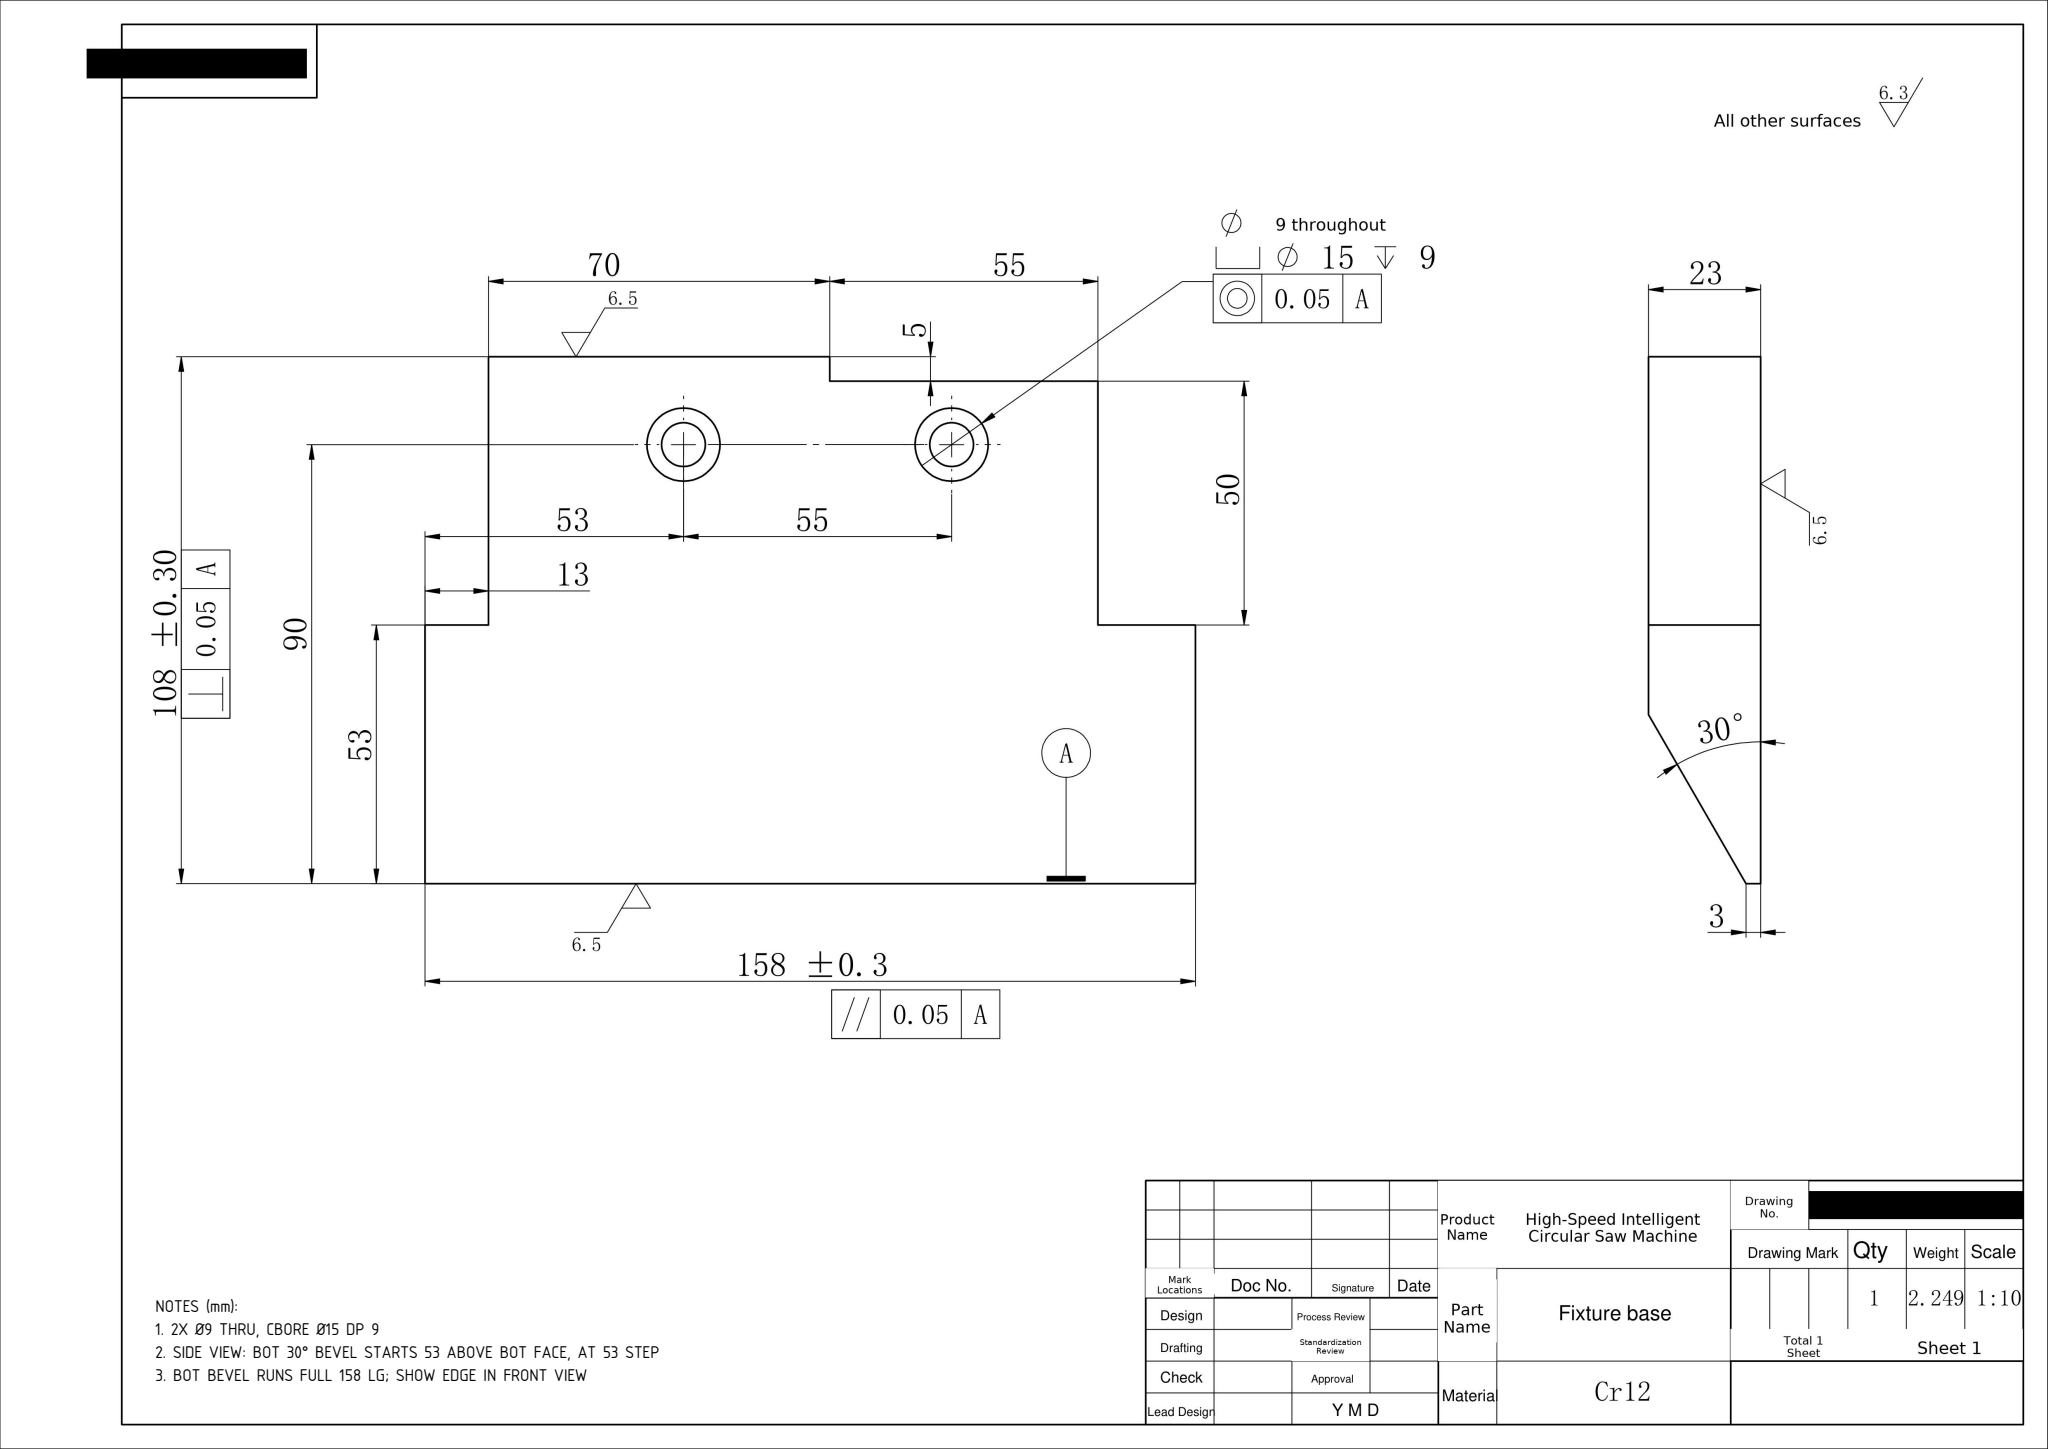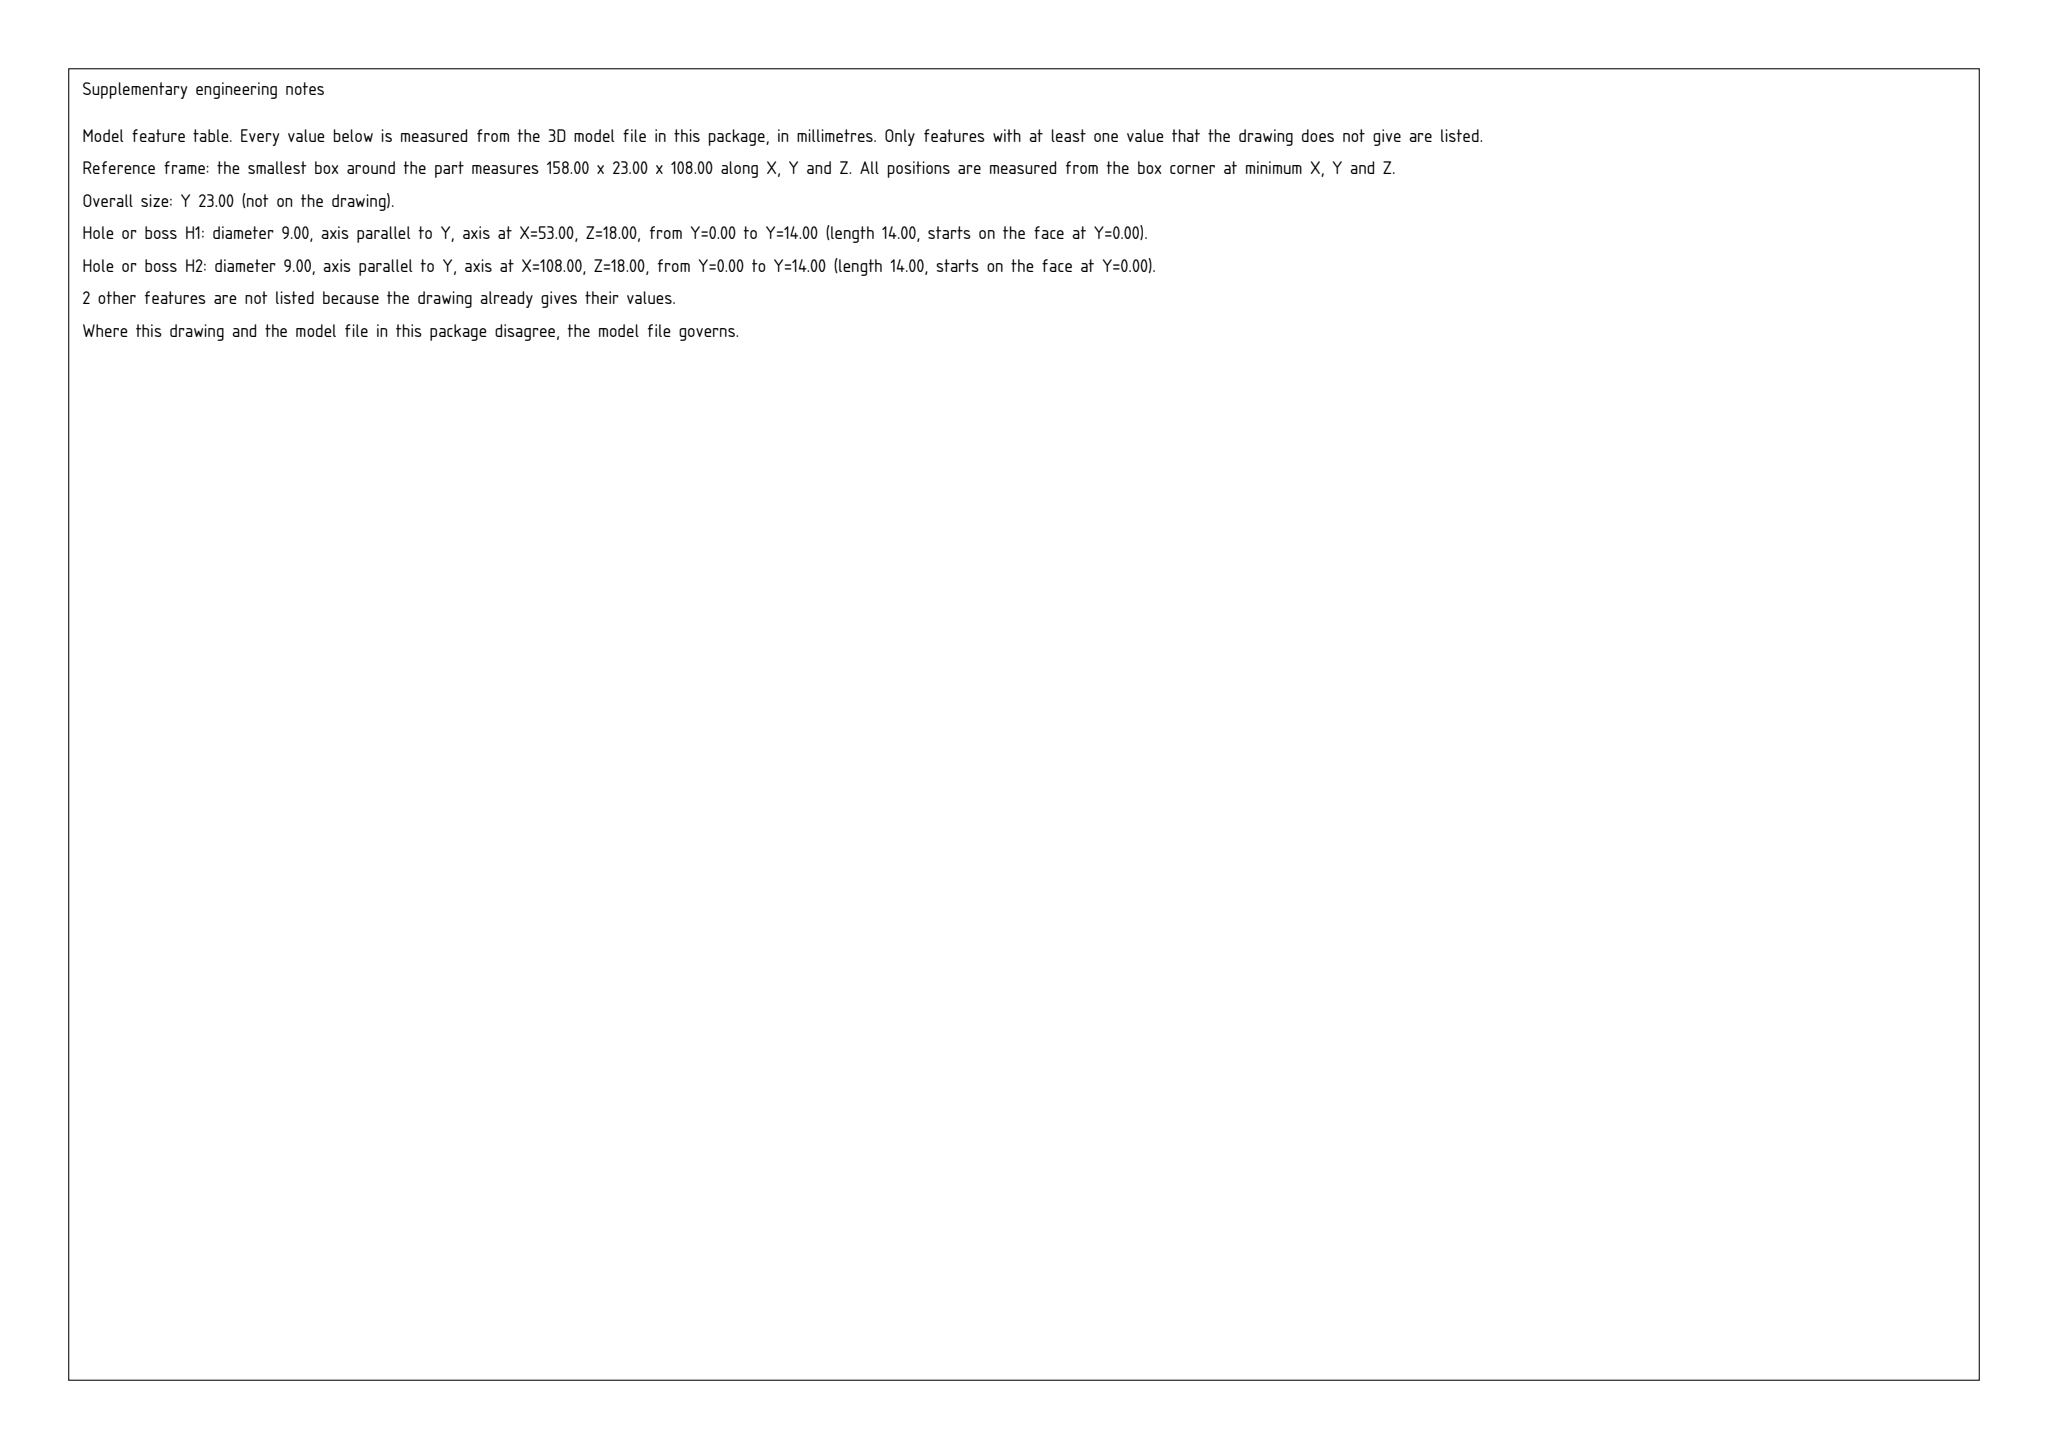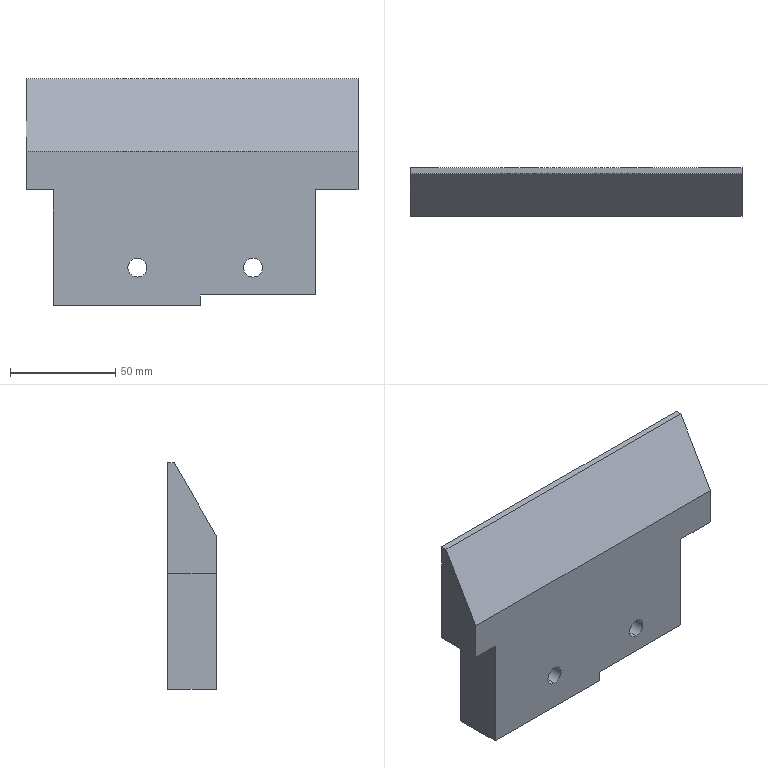Part | SolidWorks | mm | 1 solid | 23 faces | box 158 x 23 x 108 mm | volume 284707 mm3 | plane 15 | cylinder 8 | commonest cylinder face diameters 15 x4 9 x4
Drawing notes:
2X Ø9 THRU, CBORE Ø15 DP 9 | from the solid: Ø9 y-axis holes at x=53 & x=108 (55 apart), z=18; Ø15 c'bores 9 deep at same axes
SIDE VIEW: BOT 30° BEVEL STARTS 53 ABOVE BOT FACE, AT 53 STEP | from the solid: z-planes at 0,5,55,108; bevel start edge at z=55 (2 faces) = 108-55 = 53 from bottom face (z=108); matches front-view 53 step
BOT BEVEL RUNS FULL 158 LG; SHOW EDGE IN FRONT VIEW | from the solid: x-planes only at 0,13,83,138,158; no intermediate x boundary limits bevel, so it spans full 158 bbox length
build123d program:
from build123d import *

# Parameters (mm, degrees)
SKETCH2_W                                          = 125
SKETCH2_H                                          = 23
BOSS_EXTRUDE1_DEPTH                                = 210
SKETCH4_W                                          = 127
SKETCH4_H                                          = 23
CUT_EXTRUDE2_DEPTH                                 = 7
CUT_EXTRUDE3_DEPTH                                 = 234.728
SKETCH12_W                                         = 68
SKETCH12_H                                         = 28
CUT_EXTRUDE4_DEPTH                                 = 2
HOLE_SIZE_ACCORDING_TO_THE_TYPE_OF_HEX_D           = 9
HOLE_SIZE_ACCORDING_TO_THE_TYPE_OF_HEX_CBORE_D     = 15
HOLE_SIZE_ACCORDING_TO_THE_TYPE_OF_HEX_CBORE_DEPTH = 9
CUT_EXTRUDE5_DEPTH                                 = 86


with BuildPart() as part:
    # Sketch2 → Boss-Extrude1 (new body)
    with BuildSketch(Plane(origin=(0, 0, 0), x_dir=(0, 0, -1), z_dir=(1, 0, 0))):
        with Locations((37.5, 11.5)):
            Rectangle(SKETCH2_W, SKETCH2_H)
    extrude(amount=-BOSS_EXTRUDE1_DEPTH)

    # Sketch4 → Cut-Extrude2 (cut)
    with BuildSketch(Plane(origin=(0, 0, -100), x_dir=(-1, 0, 0), z_dir=(0, 0, -1))):
        with Locations((63.5, 11.5)):
            Rectangle(SKETCH4_W, SKETCH4_H)
    extrude(amount=-CUT_EXTRUDE2_DEPTH, mode=Mode.SUBTRACT)

    # Sketch9 → Cut-Extrude3 (cut, through all)
    with BuildSketch(Plane(origin=(0, 0, 0), x_dir=(0, 0, -1), z_dir=(1, 0, 0))):
        Polygon((-25, 23), (-25, 0), (24.641, 0), (-10, 20), (-10, 23), align=None)
    extrude(amount=-CUT_EXTRUDE3_DEPTH, mode=Mode.SUBTRACT)

    # Sketch12 → Cut-Extrude4 (cut)
    with BuildSketch(Plane(origin=(0, 0, -100), x_dir=(-1, 0, 0), z_dir=(0, 0, -1))):
        with Locations((161, 14)):
            Rectangle(SKETCH12_W, SKETCH12_H)
    extrude(amount=-CUT_EXTRUDE4_DEPTH, mode=Mode.SUBTRACT)

    # Hole Size _according to_ the type of Hex (through all)
    with Locations(Plane(origin=(0, 23, 0), x_dir=(1, 0, 0), z_dir=(0, 1, 0))):
        with Locations((-157, 80), (-102, 80)):
            CounterBoreHole(HOLE_SIZE_ACCORDING_TO_THE_TYPE_OF_HEX_D / 2, HOLE_SIZE_ACCORDING_TO_THE_TYPE_OF_HEX_CBORE_D / 2, HOLE_SIZE_ACCORDING_TO_THE_TYPE_OF_HEX_CBORE_DEPTH)

    # Sketch16 → Cut-Extrude5 (cut)
    with BuildSketch(Plane(origin=(0, 23, 0), x_dir=(1, 0, 0), z_dir=(0, 1, 0))):
        Polygon((-197, 98), (-197, 43), (-210, 43), (-210, 100), (-195, 100), (-195, 98), align=None)
        Polygon((-52, 43), (-52, -25), (0, -25), (0, 43), (26.134, 43), (26.134, 98), (-72, 98), (-72, 43), align=None)
    extrude(amount=-CUT_EXTRUDE5_DEPTH, mode=Mode.SUBTRACT)


solid = part.part
STEP:
#1=CARTESIAN_POINT('',(-157.,14.,-87.5));
#2=VERTEX_POINT('',#1);
#3=CARTESIAN_POINT('',(-157.,14.,-72.5));
#4=VERTEX_POINT('',#3);
#5=CARTESIAN_POINT('',(-157.,14.,-80.));
#6=DIRECTION('',(0.,1.,0.));
#7=DIRECTION('',(0.,-0.,1.));
#8=AXIS2_PLACEMENT_3D('',#5,#6,#7);
#9=CIRCLE('',#8,7.5);
#10=EDGE_CURVE('',#2,#4,#9,.T.);
#11=ORIENTED_EDGE('',*,*,#10,.F.);
#12=CARTESIAN_POINT('',(-157.,23.,-87.5));
#13=VERTEX_POINT('',#12);
#14=CARTESIAN_POINT('',(-157.,23.,-87.5));
#15=DIRECTION('',(0.,1.,0.));
#16=VECTOR('',#15,1000.);
#17=LINE('',#14,#16);
#18=EDGE_CURVE('',#2,#13,#17,.T.);
#19=ORIENTED_EDGE('',*,*,#18,.T.);
#20=CARTESIAN_POINT('',(-157.,23.,-72.5));
#21=VERTEX_POINT('',#20);
#22=CARTESIAN_POINT('',(-157.,23.,-80.));
#23=DIRECTION('',(0.,1.,0.));
#24=DIRECTION('',(0.,0.,1.));
#25=AXIS2_PLACEMENT_3D('',#22,#23,#24);
#26=CIRCLE('',#25,7.5);
#27=EDGE_CURVE('',#13,#21,#26,.T.);
#28=ORIENTED_EDGE('',*,*,#27,.T.);
#29=CARTESIAN_POINT('',(-157.,23.,-72.5));
#30=DIRECTION('',(0.,1.,0.));
#31=VECTOR('',#30,1000.);
#32=LINE('',#29,#31);
#33=EDGE_CURVE('',#4,#21,#32,.T.);
#34=ORIENTED_EDGE('',*,*,#33,.F.);
#35=EDGE_LOOP('',(#11,#19,#28,#34));
#36=FACE_OUTER_BOUND('',#35,.T.);
#37=CARTESIAN_POINT('',(-157.,23.,-80.));
#38=DIRECTION('',(0.,1.,0.));
#39=DIRECTION('',(0.,0.,1.));
#40=AXIS2_PLACEMENT_3D('',#37,#38,#39);
#41=CYLINDRICAL_SURFACE('',#40,7.5);
#42=ADVANCED_FACE('',(#36),#41,.F.);
#43=CARTESIAN_POINT('',(-157.,-0.,-84.5));
#44=VERTEX_POINT('',#43);
#45=CARTESIAN_POINT('',(-157.,-0.,-75.5));
#46=VERTEX_POINT('',#45);
#47=CARTESIAN_POINT('',(-157.,-0.,-80.));
#48=DIRECTION('',(0.,1.,0.));
#49=DIRECTION('',(0.,-0.,1.));
#50=AXIS2_PLACEMENT_3D('',#47,#48,#49);
#51=CIRCLE('',#50,4.5);
#52=EDGE_CURVE('',#44,#46,#51,.T.);
#53=ORIENTED_EDGE('',*,*,#52,.F.);
#54=CARTESIAN_POINT('',(-157.,14.,-84.5));
#55=VERTEX_POINT('',#54);
#56=CARTESIAN_POINT('',(-157.,23.,-84.5));
#57=DIRECTION('',(0.,1.,0.));
#58=VECTOR('',#57,1000.);
#59=LINE('',#56,#58);
#60=EDGE_CURVE('',#44,#55,#59,.T.);
#61=ORIENTED_EDGE('',*,*,#60,.T.);
#62=CARTESIAN_POINT('',(-157.,14.,-75.5));
#63=VERTEX_POINT('',#62);
#64=CARTESIAN_POINT('',(-157.,14.,-80.));
#65=DIRECTION('',(0.,1.,0.));
#66=DIRECTION('',(0.,0.,1.));
#67=AXIS2_PLACEMENT_3D('',#64,#65,#66);
#68=CIRCLE('',#67,4.5);
#69=EDGE_CURVE('',#55,#63,#68,.T.);
#70=ORIENTED_EDGE('',*,*,#69,.T.);
#71=CARTESIAN_POINT('',(-157.,23.,-75.5));
#72=DIRECTION('',(0.,1.,0.));
#73=VECTOR('',#72,1000.);
#74=LINE('',#71,#73);
#75=EDGE_CURVE('',#46,#63,#74,.T.);
#76=ORIENTED_EDGE('',*,*,#75,.F.);
#77=EDGE_LOOP('',(#53,#61,#70,#76));
#78=FACE_OUTER_BOUND('',#77,.T.);
#79=CARTESIAN_POINT('',(-157.,23.,-80.));
#80=DIRECTION('',(0.,1.,0.));
#81=DIRECTION('',(0.,0.,1.));
#82=AXIS2_PLACEMENT_3D('',#79,#80,#81);
#83=CYLINDRICAL_SURFACE('',#82,4.5);
#84=ADVANCED_FACE('',(#78),#83,.F.);
#85=CARTESIAN_POINT('',(-102.,14.,-87.5));
#86=VERTEX_POINT('',#85);
#87=CARTESIAN_POINT('',(-102.,14.,-72.5));
#88=VERTEX_POINT('',#87);
#89=CARTESIAN_POINT('',(-102.,14.,-80.));
#90=DIRECTION('',(0.,1.,0.));
#91=DIRECTION('',(0.,-0.,1.));
#92=AXIS2_PLACEMENT_3D('',#89,#90,#91);
#93=CIRCLE('',#92,7.5);
#94=EDGE_CURVE('',#86,#88,#93,.T.);
#95=ORIENTED_EDGE('',*,*,#94,.F.);
#96=CARTESIAN_POINT('',(-102.,23.,-87.5));
#97=VERTEX_POINT('',#96);
#98=CARTESIAN_POINT('',(-102.,23.,-87.5));
#99=DIRECTION('',(0.,1.,0.));
#100=VECTOR('',#99,1000.);
#101=LINE('',#98,#100);
#102=EDGE_CURVE('',#86,#97,#101,.T.);
#103=ORIENTED_EDGE('',*,*,#102,.T.);
#104=CARTESIAN_POINT('',(-102.,23.,-72.5));
#105=VERTEX_POINT('',#104);
#106=CARTESIAN_POINT('',(-102.,23.,-80.));
#107=DIRECTION('',(0.,1.,0.));
#108=DIRECTION('',(0.,0.,1.));
#109=AXIS2_PLACEMENT_3D('',#106,#107,#108);
#110=CIRCLE('',#109,7.5);
#111=EDGE_CURVE('',#97,#105,#110,.T.);
#112=ORIENTED_EDGE('',*,*,#111,.T.);
#113=CARTESIAN_POINT('',(-102.,23.,-72.5));
#114=DIRECTION('',(0.,1.,0.));
#115=VECTOR('',#114,1000.);
#116=LINE('',#113,#115);
#117=EDGE_CURVE('',#88,#105,#116,.T.);
#118=ORIENTED_EDGE('',*,*,#117,.F.);
#119=EDGE_LOOP('',(#95,#103,#112,#118));
#120=FACE_OUTER_BOUND('',#119,.T.);
#121=CARTESIAN_POINT('',(-102.,23.,-80.));
#122=DIRECTION('',(0.,1.,0.));
#123=DIRECTION('',(0.,0.,1.));
#124=AXIS2_PLACEMENT_3D('',#121,#122,#123);
#125=CYLINDRICAL_SURFACE('',#124,7.5);
#126=ADVANCED_FACE('',(#120),#125,.F.);
#127=CARTESIAN_POINT('',(-102.,-0.,-84.5));
#128=VERTEX_POINT('',#127);
#129=CARTESIAN_POINT('',(-102.,-0.,-75.5));
#130=VERTEX_POINT('',#129);
#131=CARTESIAN_POINT('',(-102.,-0.,-80.));
#132=DIRECTION('',(0.,1.,0.));
#133=DIRECTION('',(0.,-0.,1.));
#134=AXIS2_PLACEMENT_3D('',#131,#132,#133);
#135=CIRCLE('',#134,4.5);
#136=EDGE_CURVE('',#128,#130,#135,.T.);
#137=ORIENTED_EDGE('',*,*,#136,.F.);
#138=CARTESIAN_POINT('',(-102.,14.,-84.5));
#139=VERTEX_POINT('',#138);
#140=CARTESIAN_POINT('',(-102.,23.,-84.5));
#141=DIRECTION('',(0.,1.,0.));
#142=VECTOR('',#141,1000.);
#143=LINE('',#140,#142);
#144=EDGE_CURVE('',#128,#139,#143,.T.);
#145=ORIENTED_EDGE('',*,*,#144,.T.);
#146=CARTESIAN_POINT('',(-102.,14.,-75.5));
#147=VERTEX_POINT('',#146);
#148=CARTESIAN_POINT('',(-102.,14.,-80.));
#149=DIRECTION('',(0.,1.,0.));
#150=DIRECTION('',(0.,0.,1.));
#151=AXIS2_PLACEMENT_3D('',#148,#149,#150);
#152=CIRCLE('',#151,4.5);
#153=EDGE_CURVE('',#139,#147,#152,.T.);
#154=ORIENTED_EDGE('',*,*,#153,.T.);
#155=CARTESIAN_POINT('',(-102.,23.,-75.5));
#156=DIRECTION('',(0.,1.,0.));
#157=VECTOR('',#156,1000.);
#158=LINE('',#155,#157);
#159=EDGE_CURVE('',#130,#147,#158,.T.);
#160=ORIENTED_EDGE('',*,*,#159,.F.);
#161=EDGE_LOOP('',(#137,#145,#154,#160));
#162=FACE_OUTER_BOUND('',#161,.T.);
#163=CARTESIAN_POINT('',(-102.,23.,-80.));
#164=DIRECTION('',(0.,1.,0.));
#165=DIRECTION('',(0.,0.,1.));
#166=AXIS2_PLACEMENT_3D('',#163,#164,#165);
#167=CYLINDRICAL_SURFACE('',#166,4.5);
#168=ADVANCED_FACE('',(#162),#167,.F.);
#169=CARTESIAN_POINT('',(-197.,23.,-98.));
#170=VERTEX_POINT('',#169);
#171=CARTESIAN_POINT('',(-127.,23.,-98.));
#172=VERTEX_POINT('',#171);
#173=CARTESIAN_POINT('',(-210.,23.,-98.));
#174=DIRECTION('',(1.,0.,0.));
#175=VECTOR('',#174,1000.);
#176=LINE('',#173,#175);
#177=EDGE_CURVE('',#170,#172,#176,.T.);
#178=ORIENTED_EDGE('',*,*,#177,.F.);
#179=CARTESIAN_POINT('',(-197.,23.,-43.));
#180=VERTEX_POINT('',#179);
#181=CARTESIAN_POINT('',(-197.,23.,-98.));
#182=DIRECTION('',(0.,0.,-1.));
#183=VECTOR('',#182,1000.);
#184=LINE('',#181,#183);
#185=EDGE_CURVE('',#180,#170,#184,.T.);
#186=ORIENTED_EDGE('',*,*,#185,.F.);
#187=CARTESIAN_POINT('',(-210.,23.,-43.));
#188=VERTEX_POINT('',#187);
#189=CARTESIAN_POINT('',(-197.,23.,-43.));
#190=DIRECTION('',(1.,0.,0.));
#191=VECTOR('',#190,1000.);
#192=LINE('',#189,#191);
#193=EDGE_CURVE('',#188,#180,#192,.T.);
#194=ORIENTED_EDGE('',*,*,#193,.F.);
#195=CARTESIAN_POINT('',(-210.,23.,10.));
#196=VERTEX_POINT('',#195);
#197=CARTESIAN_POINT('',(-210.,23.,-100.));
#198=DIRECTION('',(0.,-0.,1.));
#199=VECTOR('',#198,1000.);
#200=LINE('',#197,#199);
#201=EDGE_CURVE('',#188,#196,#200,.T.);
#202=ORIENTED_EDGE('',*,*,#201,.T.);
#203=CARTESIAN_POINT('',(-52.,23.,10.));
#204=VERTEX_POINT('',#203);
#205=CARTESIAN_POINT('',(-210.,23.,10.));
#206=DIRECTION('',(1.,0.,0.));
#207=VECTOR('',#206,1000.);
#208=LINE('',#205,#207);
#209=EDGE_CURVE('',#196,#204,#208,.T.);
#210=ORIENTED_EDGE('',*,*,#209,.T.);
#211=CARTESIAN_POINT('',(-52.,23.,-43.));
#212=VERTEX_POINT('',#211);
#213=CARTESIAN_POINT('',(-52.,23.,-43.));
#214=DIRECTION('',(0.,-0.,1.));
#215=VECTOR('',#214,1000.);
#216=LINE('',#213,#215);
#217=EDGE_CURVE('',#212,#204,#216,.T.);
#218=ORIENTED_EDGE('',*,*,#217,.F.);
#219=CARTESIAN_POINT('',(-72.,23.,-43.));
#220=VERTEX_POINT('',#219);
#221=CARTESIAN_POINT('',(-72.,23.,-43.));
#222=DIRECTION('',(1.,0.,0.));
#223=VECTOR('',#222,1000.);
#224=LINE('',#221,#223);
#225=EDGE_CURVE('',#220,#212,#224,.T.);
#226=ORIENTED_EDGE('',*,*,#225,.F.);
#227=CARTESIAN_POINT('',(-72.,23.,-93.));
#228=VERTEX_POINT('',#227);
#229=CARTESIAN_POINT('',(-72.,23.,-98.));
#230=DIRECTION('',(0.,-0.,1.));
#231=VECTOR('',#230,1000.);
#232=LINE('',#229,#231);
#233=EDGE_CURVE('',#228,#220,#232,.T.);
#234=ORIENTED_EDGE('',*,*,#233,.F.);
#235=CARTESIAN_POINT('',(-127.,23.,-93.));
#236=VERTEX_POINT('',#235);
#237=CARTESIAN_POINT('',(0.,23.,-93.));
#238=DIRECTION('',(1.,0.,0.));
#239=VECTOR('',#238,1000.);
#240=LINE('',#237,#239);
#241=EDGE_CURVE('',#236,#228,#240,.T.);
#242=ORIENTED_EDGE('',*,*,#241,.F.);
#243=CARTESIAN_POINT('',(-127.,23.,-93.));
#244=DIRECTION('',(0.,0.,-1.));
#245=VECTOR('',#244,1000.);
#246=LINE('',#243,#245);
#247=EDGE_CURVE('',#236,#172,#246,.T.);
#248=ORIENTED_EDGE('',*,*,#247,.T.);
#249=EDGE_LOOP('',(#178,#186,#194,#202,#210,#218,#226,#234,#242,#248));
#250=FACE_OUTER_BOUND('',#249,.T.);
#251=CARTESIAN_POINT('',(-157.,23.,-80.));
#252=DIRECTION('',(0.,1.,0.));
#253=DIRECTION('',(0.,0.,1.));
#254=AXIS2_PLACEMENT_3D('',#251,#252,#253);
#255=CIRCLE('',#254,7.5);
#256=EDGE_CURVE('',#21,#13,#255,.T.);
#257=ORIENTED_EDGE('',*,*,#256,.F.);
#258=ORIENTED_EDGE('',*,*,#27,.F.);
#259=EDGE_LOOP('',(#257,#258));
#260=FACE_BOUND('',#259,.T.);
#261=CARTESIAN_POINT('',(-102.,23.,-80.));
#262=DIRECTION('',(0.,1.,0.));
#263=DIRECTION('',(0.,0.,1.));
#264=AXIS2_PLACEMENT_3D('',#261,#262,#263);
#265=CIRCLE('',#264,7.5);
#266=EDGE_CURVE('',#105,#97,#265,.T.);
#267=ORIENTED_EDGE('',*,*,#266,.F.);
#268=ORIENTED_EDGE('',*,*,#111,.F.);
#269=EDGE_LOOP('',(#267,#268));
#270=FACE_BOUND('',#269,.T.);
#271=CARTESIAN_POINT('',(-210.,23.,-100.));
#272=DIRECTION('',(0.,1.,0.));
#273=DIRECTION('',(0.,-0.,1.));
#274=AXIS2_PLACEMENT_3D('',#271,#272,#273);
#275=PLANE('',#274);
#276=ADVANCED_FACE('',(#250,#260,#270),#275,.T.);
#277=CARTESIAN_POINT('',(-197.,0.,-98.));
#278=VERTEX_POINT('',#277);
#279=CARTESIAN_POINT('',(-197.,0.,-43.));
#280=VERTEX_POINT('',#279);
#281=CARTESIAN_POINT('',(-197.,0.,25.));
#282=DIRECTION('',(-0.,0.,1.));
#283=VECTOR('',#282,1000.);
#284=LINE('',#281,#283);
#285=EDGE_CURVE('',#278,#280,#284,.T.);
#286=ORIENTED_EDGE('',*,*,#285,.F.);
#287=CARTESIAN_POINT('',(-127.,0.,-98.));
#288=VERTEX_POINT('',#287);
#289=CARTESIAN_POINT('',(-127.,0.,-98.));
#290=DIRECTION('',(-1.,0.,0.));
#291=VECTOR('',#290,1000.);
#292=LINE('',#289,#291);
#293=EDGE_CURVE('',#288,#278,#292,.T.);
#294=ORIENTED_EDGE('',*,*,#293,.F.);
#295=CARTESIAN_POINT('',(-127.,0.,-93.));
#296=VERTEX_POINT('',#295);
#297=CARTESIAN_POINT('',(-127.,0.,-93.));
#298=DIRECTION('',(0.,0.,-1.));
#299=VECTOR('',#298,1000.);
#300=LINE('',#297,#299);
#301=EDGE_CURVE('',#296,#288,#300,.T.);
#302=ORIENTED_EDGE('',*,*,#301,.F.);
#303=CARTESIAN_POINT('',(-72.,0.,-93.));
#304=VERTEX_POINT('',#303);
#305=CARTESIAN_POINT('',(0.,0.,-93.));
#306=DIRECTION('',(-1.,0.,0.));
#307=VECTOR('',#306,1000.);
#308=LINE('',#305,#307);
#309=EDGE_CURVE('',#304,#296,#308,.T.);
#310=ORIENTED_EDGE('',*,*,#309,.F.);
#311=CARTESIAN_POINT('',(-72.,0.,-43.));
#312=VERTEX_POINT('',#311);
#313=CARTESIAN_POINT('',(-72.,0.,25.));
#314=DIRECTION('',(0.,0.,-1.));
#315=VECTOR('',#314,1000.);
#316=LINE('',#313,#315);
#317=EDGE_CURVE('',#312,#304,#316,.T.);
#318=ORIENTED_EDGE('',*,*,#317,.F.);
#319=CARTESIAN_POINT('',(-52.,0.,-43.));
#320=VERTEX_POINT('',#319);
#321=CARTESIAN_POINT('',(-210.,0.,-43.));
#322=DIRECTION('',(-1.,0.,-0.));
#323=VECTOR('',#322,1000.);
#324=LINE('',#321,#323);
#325=EDGE_CURVE('',#320,#312,#324,.T.);
#326=ORIENTED_EDGE('',*,*,#325,.F.);
#327=CARTESIAN_POINT('',(-52.,-0.,-24.641));
#328=VERTEX_POINT('',#327);
#329=CARTESIAN_POINT('',(-52.,0.,25.));
#330=DIRECTION('',(-0.,0.,-1.));
#331=VECTOR('',#330,1000.);
#332=LINE('',#329,#331);
#333=EDGE_CURVE('',#328,#320,#332,.T.);
#334=ORIENTED_EDGE('',*,*,#333,.F.);
#335=CARTESIAN_POINT('',(-210.,-0.,-24.641));
#336=VERTEX_POINT('',#335);
#337=CARTESIAN_POINT('',(-210.,-0.,-24.641));
#338=DIRECTION('',(1.,0.,0.));
#339=VECTOR('',#338,1000.);
#340=LINE('',#337,#339);
#341=EDGE_CURVE('',#336,#328,#340,.T.);
#342=ORIENTED_EDGE('',*,*,#341,.F.);
#343=CARTESIAN_POINT('',(-210.,0.,-43.));
#344=VERTEX_POINT('',#343);
#345=CARTESIAN_POINT('',(-210.,0.,25.));
#346=DIRECTION('',(0.,0.,-1.));
#347=VECTOR('',#346,1000.);
#348=LINE('',#345,#347);
#349=EDGE_CURVE('',#336,#344,#348,.T.);
#350=ORIENTED_EDGE('',*,*,#349,.T.);
#351=CARTESIAN_POINT('',(-210.,0.,-43.));
#352=DIRECTION('',(-1.,0.,-0.));
#353=VECTOR('',#352,1000.);
#354=LINE('',#351,#353);
#355=EDGE_CURVE('',#280,#344,#354,.T.);
#356=ORIENTED_EDGE('',*,*,#355,.F.);
#357=EDGE_LOOP('',(#286,#294,#302,#310,#318,#326,#334,#342,#350,#356));
#358=FACE_OUTER_BOUND('',#357,.T.);
#359=CARTESIAN_POINT('',(-157.,-0.,-80.));
#360=DIRECTION('',(0.,1.,0.));
#361=DIRECTION('',(0.,-0.,1.));
#362=AXIS2_PLACEMENT_3D('',#359,#360,#361);
#363=CIRCLE('',#362,4.5);
#364=EDGE_CURVE('',#46,#44,#363,.T.);
#365=ORIENTED_EDGE('',*,*,#364,.T.);
#366=ORIENTED_EDGE('',*,*,#52,.T.);
#367=EDGE_LOOP('',(#365,#366));
#368=FACE_BOUND('',#367,.T.);
#369=CARTESIAN_POINT('',(-102.,-0.,-80.));
#370=DIRECTION('',(0.,1.,0.));
#371=DIRECTION('',(0.,-0.,1.));
#372=AXIS2_PLACEMENT_3D('',#369,#370,#371);
#373=CIRCLE('',#372,4.5);
#374=EDGE_CURVE('',#130,#128,#373,.T.);
#375=ORIENTED_EDGE('',*,*,#374,.T.);
#376=ORIENTED_EDGE('',*,*,#136,.T.);
#377=EDGE_LOOP('',(#375,#376));
#378=FACE_BOUND('',#377,.T.);
#379=CARTESIAN_POINT('',(-210.,0.,25.));
#380=DIRECTION('',(0.,-1.,0.));
#381=DIRECTION('',(0.,0.,-1.));
#382=AXIS2_PLACEMENT_3D('',#379,#380,#381);
#383=PLANE('',#382);
#384=ADVANCED_FACE('',(#358,#368,#378),#383,.T.);
#385=ORIENTED_EDGE('',*,*,#201,.F.);
#386=CARTESIAN_POINT('',(-210.,0.,-43.));
#387=DIRECTION('',(0.,-1.,-0.));
#388=VECTOR('',#387,1000.);
#389=LINE('',#386,#388);
#390=EDGE_CURVE('',#188,#344,#389,.T.);
#391=ORIENTED_EDGE('',*,*,#390,.T.);
#392=ORIENTED_EDGE('',*,*,#349,.F.);
#393=CARTESIAN_POINT('',(-210.,20.,10.));
#394=VERTEX_POINT('',#393);
#395=CARTESIAN_POINT('',(-210.,20.,10.));
#396=DIRECTION('',(0.,0.5,0.866));
#397=VECTOR('',#396,1000.);
#398=LINE('',#395,#397);
#399=EDGE_CURVE('',#336,#394,#398,.T.);
#400=ORIENTED_EDGE('',*,*,#399,.T.);
#401=CARTESIAN_POINT('',(-210.,20.,10.));
#402=DIRECTION('',(0.,1.,0.));
#403=VECTOR('',#402,1000.);
#404=LINE('',#401,#403);
#405=EDGE_CURVE('',#394,#196,#404,.T.);
#406=ORIENTED_EDGE('',*,*,#405,.T.);
#407=EDGE_LOOP('',(#385,#391,#392,#400,#406));
#408=FACE_OUTER_BOUND('',#407,.T.);
#409=CARTESIAN_POINT('',(-210.,0.,0.));
#410=DIRECTION('',(1.,0.,0.));
#411=DIRECTION('',(0.,0.,-1.));
#412=AXIS2_PLACEMENT_3D('',#409,#410,#411);
#413=PLANE('',#412);
#414=ADVANCED_FACE('',(#408),#413,.F.);
#415=ORIENTED_EDGE('',*,*,#301,.T.);
#416=CARTESIAN_POINT('',(-127.,23.,-98.));
#417=DIRECTION('',(0.,1.,0.));
#418=VECTOR('',#417,1000.);
#419=LINE('',#416,#418);
#420=EDGE_CURVE('',#288,#172,#419,.T.);
#421=ORIENTED_EDGE('',*,*,#420,.T.);
#422=ORIENTED_EDGE('',*,*,#247,.F.);
#423=CARTESIAN_POINT('',(-127.,23.,-93.));
#424=DIRECTION('',(0.,1.,0.));
#425=VECTOR('',#424,1000.);
#426=LINE('',#423,#425);
#427=EDGE_CURVE('',#296,#236,#426,.T.);
#428=ORIENTED_EDGE('',*,*,#427,.F.);
#429=EDGE_LOOP('',(#415,#421,#422,#428));
#430=FACE_OUTER_BOUND('',#429,.T.);
#431=CARTESIAN_POINT('',(-127.,23.,-93.));
#432=DIRECTION('',(-1.,0.,0.));
#433=DIRECTION('',(0.,0.,1.));
#434=AXIS2_PLACEMENT_3D('',#431,#432,#433);
#435=PLANE('',#434);
#436=ADVANCED_FACE('',(#430),#435,.F.);
#437=CARTESIAN_POINT('',(-72.,0.,-93.));
#438=DIRECTION('',(0.,1.,0.));
#439=VECTOR('',#438,1000.);
#440=LINE('',#437,#439);
#441=EDGE_CURVE('',#304,#228,#440,.T.);
#442=ORIENTED_EDGE('',*,*,#441,.F.);
#443=ORIENTED_EDGE('',*,*,#309,.T.);
#444=ORIENTED_EDGE('',*,*,#427,.T.);
#445=ORIENTED_EDGE('',*,*,#241,.T.);
#446=EDGE_LOOP('',(#442,#443,#444,#445));
#447=FACE_OUTER_BOUND('',#446,.T.);
#448=CARTESIAN_POINT('',(0.,0.,-93.));
#449=DIRECTION('',(0.,0.,-1.));
#450=DIRECTION('',(-1.,0.,0.));
#451=AXIS2_PLACEMENT_3D('',#448,#449,#450);
#452=PLANE('',#451);
#453=ADVANCED_FACE('',(#447),#452,.T.);
#454=ORIENTED_EDGE('',*,*,#341,.T.);
#455=CARTESIAN_POINT('',(-52.,20.,10.));
#456=VERTEX_POINT('',#455);
#457=CARTESIAN_POINT('',(-52.,20.,10.));
#458=DIRECTION('',(0.,0.5,0.866));
#459=VECTOR('',#458,1000.);
#460=LINE('',#457,#459);
#461=EDGE_CURVE('',#328,#456,#460,.T.);
#462=ORIENTED_EDGE('',*,*,#461,.T.);
#463=CARTESIAN_POINT('',(-210.,20.,10.));
#464=DIRECTION('',(1.,0.,0.));
#465=VECTOR('',#464,1000.);
#466=LINE('',#463,#465);
#467=EDGE_CURVE('',#394,#456,#466,.T.);
#468=ORIENTED_EDGE('',*,*,#467,.F.);
#469=ORIENTED_EDGE('',*,*,#399,.F.);
#470=EDGE_LOOP('',(#454,#462,#468,#469));
#471=FACE_OUTER_BOUND('',#470,.T.);
#472=CARTESIAN_POINT('',(-210.,20.,10.));
#473=DIRECTION('',(0.,0.866,-0.5));
#474=DIRECTION('',(0.,0.5,0.866));
#475=AXIS2_PLACEMENT_3D('',#472,#473,#474);
#476=PLANE('',#475);
#477=ADVANCED_FACE('',(#471),#476,.F.);
#478=ORIENTED_EDGE('',*,*,#467,.T.);
#479=CARTESIAN_POINT('',(-52.,20.,10.));
#480=DIRECTION('',(-0.,1.,0.));
#481=VECTOR('',#480,1000.);
#482=LINE('',#479,#481);
#483=EDGE_CURVE('',#456,#204,#482,.T.);
#484=ORIENTED_EDGE('',*,*,#483,.T.);
#485=ORIENTED_EDGE('',*,*,#209,.F.);
#486=ORIENTED_EDGE('',*,*,#405,.F.);
#487=EDGE_LOOP('',(#478,#484,#485,#486));
#488=FACE_OUTER_BOUND('',#487,.T.);
#489=CARTESIAN_POINT('',(-210.,20.,10.));
#490=DIRECTION('',(0.,0.,-1.));
#491=DIRECTION('',(-1.,0.,0.));
#492=AXIS2_PLACEMENT_3D('',#489,#490,#491);
#493=PLANE('',#492);
#494=ADVANCED_FACE('',(#488),#493,.F.);
#495=ORIENTED_EDGE('',*,*,#177,.T.);
#496=ORIENTED_EDGE('',*,*,#420,.F.);
#497=ORIENTED_EDGE('',*,*,#293,.T.);
#498=CARTESIAN_POINT('',(-197.,-63.,-98.));
#499=DIRECTION('',(0.,1.,0.));
#500=VECTOR('',#499,1000.);
#501=LINE('',#498,#500);
#502=EDGE_CURVE('',#278,#170,#501,.T.);
#503=ORIENTED_EDGE('',*,*,#502,.T.);
#504=EDGE_LOOP('',(#495,#496,#497,#503));
#505=FACE_OUTER_BOUND('',#504,.T.);
#506=CARTESIAN_POINT('',(0.,0.,-98.));
#507=DIRECTION('',(0.,0.,1.));
#508=DIRECTION('',(1.,0.,0.));
#509=AXIS2_PLACEMENT_3D('',#506,#507,#508);
#510=PLANE('',#509);
#511=ADVANCED_FACE('',(#505),#510,.F.);
#512=ORIENTED_EDGE('',*,*,#144,.F.);
#513=ORIENTED_EDGE('',*,*,#374,.F.);
#514=ORIENTED_EDGE('',*,*,#159,.T.);
#515=CARTESIAN_POINT('',(-102.,14.,-80.));
#516=DIRECTION('',(0.,1.,0.));
#517=DIRECTION('',(0.,0.,1.));
#518=AXIS2_PLACEMENT_3D('',#515,#516,#517);
#519=CIRCLE('',#518,4.5);
#520=EDGE_CURVE('',#147,#139,#519,.T.);
#521=ORIENTED_EDGE('',*,*,#520,.T.);
#522=EDGE_LOOP('',(#512,#513,#514,#521));
#523=FACE_OUTER_BOUND('',#522,.T.);
#524=CARTESIAN_POINT('',(-102.,23.,-80.));
#525=DIRECTION('',(0.,1.,0.));
#526=DIRECTION('',(0.,0.,1.));
#527=AXIS2_PLACEMENT_3D('',#524,#525,#526);
#528=CYLINDRICAL_SURFACE('',#527,4.5);
#529=ADVANCED_FACE('',(#523),#528,.F.);
#530=ORIENTED_EDGE('',*,*,#520,.F.);
#531=ORIENTED_EDGE('',*,*,#153,.F.);
#532=EDGE_LOOP('',(#530,#531));
#533=FACE_BOUND('',#532,.T.);
#534=CARTESIAN_POINT('',(-102.,14.,-80.));
#535=DIRECTION('',(0.,1.,0.));
#536=DIRECTION('',(0.,-0.,1.));
#537=AXIS2_PLACEMENT_3D('',#534,#535,#536);
#538=CIRCLE('',#537,7.5);
#539=EDGE_CURVE('',#88,#86,#538,.T.);
#540=ORIENTED_EDGE('',*,*,#539,.T.);
#541=ORIENTED_EDGE('',*,*,#94,.T.);
#542=EDGE_LOOP('',(#540,#541));
#543=FACE_OUTER_BOUND('',#542,.T.);
#544=CARTESIAN_POINT('',(-97.5,14.,-80.));
#545=DIRECTION('',(0.,-1.,-0.));
#546=DIRECTION('',(0.,0.,-1.));
#547=AXIS2_PLACEMENT_3D('',#544,#545,#546);
#548=PLANE('',#547);
#549=ADVANCED_FACE('',(#533,#543),#548,.F.);
#550=ORIENTED_EDGE('',*,*,#102,.F.);
#551=ORIENTED_EDGE('',*,*,#539,.F.);
#552=ORIENTED_EDGE('',*,*,#117,.T.);
#553=ORIENTED_EDGE('',*,*,#266,.T.);
#554=EDGE_LOOP('',(#550,#551,#552,#553));
#555=FACE_OUTER_BOUND('',#554,.T.);
#556=CARTESIAN_POINT('',(-102.,23.,-80.));
#557=DIRECTION('',(0.,1.,0.));
#558=DIRECTION('',(0.,0.,1.));
#559=AXIS2_PLACEMENT_3D('',#556,#557,#558);
#560=CYLINDRICAL_SURFACE('',#559,7.5);
#561=ADVANCED_FACE('',(#555),#560,.F.);
#562=ORIENTED_EDGE('',*,*,#60,.F.);
#563=ORIENTED_EDGE('',*,*,#364,.F.);
#564=ORIENTED_EDGE('',*,*,#75,.T.);
#565=CARTESIAN_POINT('',(-157.,14.,-80.));
#566=DIRECTION('',(0.,1.,0.));
#567=DIRECTION('',(0.,0.,1.));
#568=AXIS2_PLACEMENT_3D('',#565,#566,#567);
#569=CIRCLE('',#568,4.5);
#570=EDGE_CURVE('',#63,#55,#569,.T.);
#571=ORIENTED_EDGE('',*,*,#570,.T.);
#572=EDGE_LOOP('',(#562,#563,#564,#571));
#573=FACE_OUTER_BOUND('',#572,.T.);
#574=CARTESIAN_POINT('',(-157.,23.,-80.));
#575=DIRECTION('',(0.,1.,0.));
#576=DIRECTION('',(0.,0.,1.));
#577=AXIS2_PLACEMENT_3D('',#574,#575,#576);
#578=CYLINDRICAL_SURFACE('',#577,4.5);
#579=ADVANCED_FACE('',(#573),#578,.F.);
#580=ORIENTED_EDGE('',*,*,#570,.F.);
#581=ORIENTED_EDGE('',*,*,#69,.F.);
#582=EDGE_LOOP('',(#580,#581));
#583=FACE_BOUND('',#582,.T.);
#584=CARTESIAN_POINT('',(-157.,14.,-80.));
#585=DIRECTION('',(0.,1.,0.));
#586=DIRECTION('',(0.,-0.,1.));
#587=AXIS2_PLACEMENT_3D('',#584,#585,#586);
#588=CIRCLE('',#587,7.5);
#589=EDGE_CURVE('',#4,#2,#588,.T.);
#590=ORIENTED_EDGE('',*,*,#589,.T.);
#591=ORIENTED_EDGE('',*,*,#10,.T.);
#592=EDGE_LOOP('',(#590,#591));
#593=FACE_OUTER_BOUND('',#592,.T.);
#594=CARTESIAN_POINT('',(-152.5,14.,-80.));
#595=DIRECTION('',(0.,-1.,-0.));
#596=DIRECTION('',(0.,0.,-1.));
#597=AXIS2_PLACEMENT_3D('',#594,#595,#596);
#598=PLANE('',#597);
#599=ADVANCED_FACE('',(#583,#593),#598,.F.);
#600=ORIENTED_EDGE('',*,*,#18,.F.);
#601=ORIENTED_EDGE('',*,*,#589,.F.);
#602=ORIENTED_EDGE('',*,*,#33,.T.);
#603=ORIENTED_EDGE('',*,*,#256,.T.);
#604=EDGE_LOOP('',(#600,#601,#602,#603));
#605=FACE_OUTER_BOUND('',#604,.T.);
#606=CARTESIAN_POINT('',(-157.,23.,-80.));
#607=DIRECTION('',(0.,1.,0.));
#608=DIRECTION('',(0.,0.,1.));
#609=AXIS2_PLACEMENT_3D('',#606,#607,#608);
#610=CYLINDRICAL_SURFACE('',#609,7.5);
#611=ADVANCED_FACE('',(#605),#610,.F.);
#612=ORIENTED_EDGE('',*,*,#285,.T.);
#613=CARTESIAN_POINT('',(-197.,-63.,-43.));
#614=DIRECTION('',(0.,1.,0.));
#615=VECTOR('',#614,1000.);
#616=LINE('',#613,#615);
#617=EDGE_CURVE('',#280,#180,#616,.T.);
#618=ORIENTED_EDGE('',*,*,#617,.T.);
#619=ORIENTED_EDGE('',*,*,#185,.T.);
#620=ORIENTED_EDGE('',*,*,#502,.F.);
#621=EDGE_LOOP('',(#612,#618,#619,#620));
#622=FACE_OUTER_BOUND('',#621,.T.);
#623=CARTESIAN_POINT('',(-197.,-63.,-98.));
#624=DIRECTION('',(1.,-0.,0.));
#625=DIRECTION('',(0.,0.,-1.));
#626=AXIS2_PLACEMENT_3D('',#623,#624,#625);
#627=PLANE('',#626);
#628=ADVANCED_FACE('',(#622),#627,.F.);
#629=ORIENTED_EDGE('',*,*,#355,.T.);
#630=ORIENTED_EDGE('',*,*,#390,.F.);
#631=ORIENTED_EDGE('',*,*,#193,.T.);
#632=ORIENTED_EDGE('',*,*,#617,.F.);
#633=EDGE_LOOP('',(#629,#630,#631,#632));
#634=FACE_OUTER_BOUND('',#633,.T.);
#635=CARTESIAN_POINT('',(-197.,-63.,-43.));
#636=DIRECTION('',(-0.,-0.,1.));
#637=DIRECTION('',(1.,0.,0.));
#638=AXIS2_PLACEMENT_3D('',#635,#636,#637);
#639=PLANE('',#638);
#640=ADVANCED_FACE('',(#634),#639,.F.);
#641=ORIENTED_EDGE('',*,*,#317,.T.);
#642=ORIENTED_EDGE('',*,*,#441,.T.);
#643=ORIENTED_EDGE('',*,*,#233,.T.);
#644=CARTESIAN_POINT('',(-72.,-63.,-43.));
#645=DIRECTION('',(0.,1.,0.));
#646=VECTOR('',#645,1000.);
#647=LINE('',#644,#646);
#648=EDGE_CURVE('',#312,#220,#647,.T.);
#649=ORIENTED_EDGE('',*,*,#648,.F.);
#650=EDGE_LOOP('',(#641,#642,#643,#649));
#651=FACE_OUTER_BOUND('',#650,.T.);
#652=CARTESIAN_POINT('',(-72.,-63.,-98.));
#653=DIRECTION('',(-1.,0.,0.));
#654=DIRECTION('',(0.,0.,1.));
#655=AXIS2_PLACEMENT_3D('',#652,#653,#654);
#656=PLANE('',#655);
#657=ADVANCED_FACE('',(#651),#656,.F.);
#658=ORIENTED_EDGE('',*,*,#333,.T.);
#659=CARTESIAN_POINT('',(-52.,-63.,-43.));
#660=DIRECTION('',(0.,1.,0.));
#661=VECTOR('',#660,1000.);
#662=LINE('',#659,#661);
#663=EDGE_CURVE('',#320,#212,#662,.T.);
#664=ORIENTED_EDGE('',*,*,#663,.T.);
#665=ORIENTED_EDGE('',*,*,#217,.T.);
#666=ORIENTED_EDGE('',*,*,#483,.F.);
#667=ORIENTED_EDGE('',*,*,#461,.F.);
#668=EDGE_LOOP('',(#658,#664,#665,#666,#667));
#669=FACE_OUTER_BOUND('',#668,.T.);
#670=CARTESIAN_POINT('',(-52.,-63.,-43.));
#671=DIRECTION('',(-1.,-0.,0.));
#672=DIRECTION('',(0.,0.,1.));
#673=AXIS2_PLACEMENT_3D('',#670,#671,#672);
#674=PLANE('',#673);
#675=ADVANCED_FACE('',(#669),#674,.F.);
#676=ORIENTED_EDGE('',*,*,#325,.T.);
#677=ORIENTED_EDGE('',*,*,#648,.T.);
#678=ORIENTED_EDGE('',*,*,#225,.T.);
#679=ORIENTED_EDGE('',*,*,#663,.F.);
#680=EDGE_LOOP('',(#676,#677,#678,#679));
#681=FACE_OUTER_BOUND('',#680,.T.);
#682=CARTESIAN_POINT('',(-72.,-63.,-43.));
#683=DIRECTION('',(-0.,-0.,1.));
#684=DIRECTION('',(1.,0.,0.));
#685=AXIS2_PLACEMENT_3D('',#682,#683,#684);
#686=PLANE('',#685);
#687=ADVANCED_FACE('',(#681),#686,.F.);
#688=CLOSED_SHELL('',(#42,#84,#126,#168,#276,#384,#414,#436,#453,#477,#494,#511,#529,#549,#561,#579,#599,#611,#628,#640,#657,#675,#687));
#689=MANIFOLD_SOLID_BREP('',#688);
#690=CARTESIAN_POINT('',(0.,0.,0.));
#691=DIRECTION('',(0.,0.,1.));
#692=DIRECTION('',(1.,0.,0.));
#693=AXIS2_PLACEMENT_3D('',#690,#691,#692);
#694=(LENGTH_UNIT()NAMED_UNIT(*)SI_UNIT(.MILLI.,.METRE.));
#695=UNCERTAINTY_MEASURE_WITH_UNIT(LENGTH_MEASURE(0.00001),#694,'','');
#696=(NAMED_UNIT(*)PLANE_ANGLE_UNIT()SI_UNIT($,.RADIAN.));
#697=(NAMED_UNIT(*)SI_UNIT($,.STERADIAN.)SOLID_ANGLE_UNIT());
#698=(GEOMETRIC_REPRESENTATION_CONTEXT(3)GLOBAL_UNCERTAINTY_ASSIGNED_CONTEXT((#695))GLOBAL_UNIT_ASSIGNED_CONTEXT((#694,#696,#697))REPRESENTATION_CONTEXT('',''));
#699=ADVANCED_BREP_SHAPE_REPRESENTATION('',(#689,#693),#698);